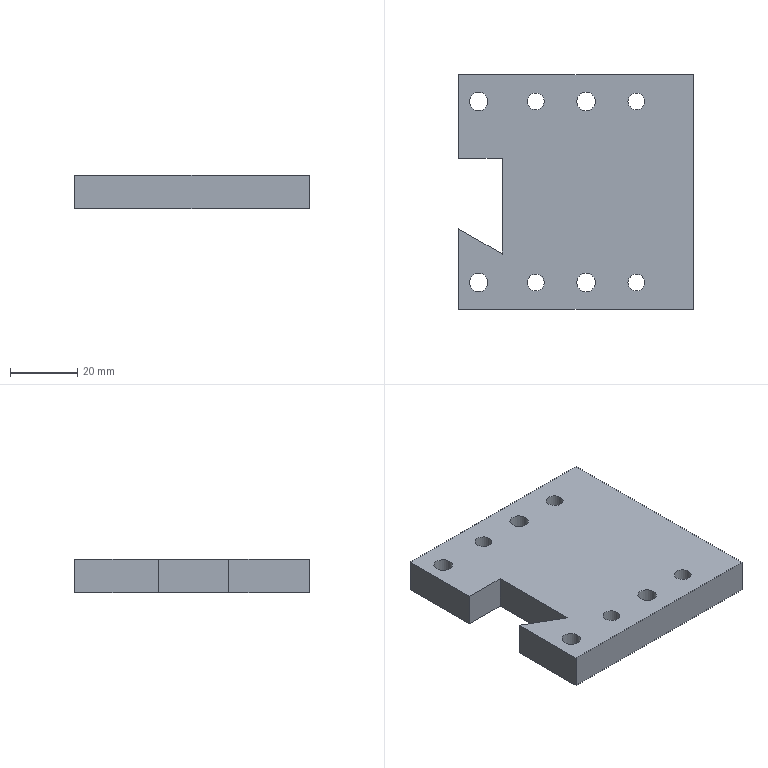Component | NX | BASE_PLATE | 1 solid | 26 faces | volume 42864 mm3 | plane 14 | cylinder 12 | commonest cylinder face diameters 5.5 x4 10 x4 5 x4